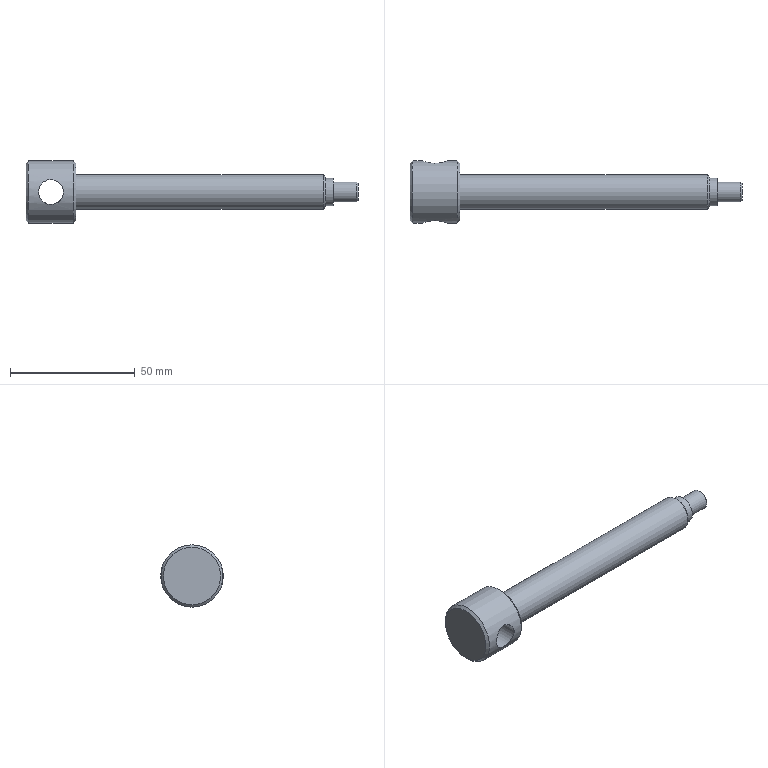Component | NX | SCREW_ROD | 1 solid | 14 faces | box 133 x 25 x 25 mm | volume 23976 mm3 | cylinder 5 | plane 5 | cone 4 | commonest cylinder face diameters 25 x1 8 x1 11 x1 14 x1 10 x1
STEP:
#1=CARTESIAN_POINT('',(0.,0.,0.));
#2=DIRECTION('',(0.,0.,1.));
#3=DIRECTION('',(1.,0.,0.));
#4=AXIS2_PLACEMENT_3D('',#1,#2,#3);
#5=CARTESIAN_POINT('',(-201.627,0.,27.5));
#6=VERTEX_POINT('',#5);
#7=CARTESIAN_POINT('',(-201.627,0.,15.));
#8=DIRECTION('',(1.,0.,0.));
#9=DIRECTION('',(0.,0.,1.));
#10=AXIS2_PLACEMENT_3D('',#7,#8,#9);
#11=CIRCLE('',#10,12.5);
#12=CARTESIAN_POINT('',(-182.627,0.,15.));
#13=DIRECTION('',(-1.,0.,0.));
#14=DIRECTION('',(0.,0.,1.));
#15=AXIS2_PLACEMENT_3D('',#12,#13,#14);
#16=CYLINDRICAL_SURFACE('',#15,12.5);
#17=CARTESIAN_POINT('',(6.283,19.));
#18=DIRECTION('',(-1.,0.));
#19=VECTOR('',#18,1.);
#20=LINE('',#17,#19);
#21=(GEOMETRIC_REPRESENTATION_CONTEXT(2)PARAMETRIC_REPRESENTATION_CONTEXT()REPRESENTATION_CONTEXT('',''));
#22=DEFINITIONAL_REPRESENTATION('',(#20),#21);
#23=PCURVE('',#16,#22);
#24=CARTESIAN_POINT('',(-201.627,0.,15.));
#25=DIRECTION('',(1.,0.,0.));
#26=DIRECTION('',(0.,0.,-1.));
#27=AXIS2_PLACEMENT_3D('',#24,#25,#26);
#28=CONICAL_SURFACE('',#27,12.5,0.7854);
#29=CARTESIAN_POINT('',(3.142,0.));
#30=DIRECTION('',(1.,0.));
#31=VECTOR('',#30,1.);
#32=LINE('',#29,#31);
#33=(GEOMETRIC_REPRESENTATION_CONTEXT(2)PARAMETRIC_REPRESENTATION_CONTEXT()REPRESENTATION_CONTEXT('',''));
#34=DEFINITIONAL_REPRESENTATION('',(#32),#33);
#35=PCURVE('',#28,#34);
#36=SURFACE_CURVE('',#11,(#23,#35),.PCURVE_S1.);
#37=EDGE_CURVE('',#6,#6,#36,.T.);
#38=ORIENTED_EDGE('',*,*,#37,.T.);
#39=CARTESIAN_POINT('',(-183.627,-0.,27.5));
#40=VERTEX_POINT('',#39);
#41=CARTESIAN_POINT('',(-183.627,-0.,27.5));
#42=CARTESIAN_POINT('',(-201.627,-0.,27.5));
#43=B_SPLINE_CURVE_WITH_KNOTS('',1,(#41,#42),.UNSPECIFIED.,.F.,.F.,(2,2),(1.,19.),.PIECEWISE_BEZIER_KNOTS.);
#44=CARTESIAN_POINT('',(0.,0.));
#45=DIRECTION('',(0.,1.));
#46=VECTOR('',#45,1.);
#47=LINE('',#44,#46);
#48=(GEOMETRIC_REPRESENTATION_CONTEXT(2)PARAMETRIC_REPRESENTATION_CONTEXT()REPRESENTATION_CONTEXT('',''));
#49=DEFINITIONAL_REPRESENTATION('',(#47),#48);
#50=PCURVE('',#16,#49);
#51=CARTESIAN_POINT('',(6.283,0.));
#52=DIRECTION('',(0.,1.));
#53=VECTOR('',#52,1.);
#54=LINE('',#51,#53);
#55=(GEOMETRIC_REPRESENTATION_CONTEXT(2)PARAMETRIC_REPRESENTATION_CONTEXT()REPRESENTATION_CONTEXT('',''));
#56=DEFINITIONAL_REPRESENTATION('',(#54),#55);
#57=PCURVE('',#16,#56);
#58=SEAM_CURVE('',#43,(#50,#57),.PCURVE_S1.);
#59=EDGE_CURVE('',#40,#6,#58,.T.);
#60=ORIENTED_EDGE('',*,*,#59,.F.);
#61=CARTESIAN_POINT('',(-183.627,0.,2.5));
#62=VERTEX_POINT('',#61);
#63=CARTESIAN_POINT('',(-183.627,0.,15.));
#64=DIRECTION('',(-1.,0.,0.));
#65=DIRECTION('',(0.,0.,-1.));
#66=AXIS2_PLACEMENT_3D('',#63,#64,#65);
#67=CIRCLE('',#66,12.5);
#68=CARTESIAN_POINT('',(-3.142,1.));
#69=DIRECTION('',(1.,0.));
#70=VECTOR('',#69,1.);
#71=LINE('',#68,#70);
#72=(GEOMETRIC_REPRESENTATION_CONTEXT(2)PARAMETRIC_REPRESENTATION_CONTEXT()REPRESENTATION_CONTEXT('',''));
#73=DEFINITIONAL_REPRESENTATION('',(#71),#72);
#74=PCURVE('',#16,#73);
#75=CARTESIAN_POINT('',(-183.627,0.,15.));
#76=DIRECTION('',(-1.,0.,0.));
#77=DIRECTION('',(0.,0.,1.));
#78=AXIS2_PLACEMENT_3D('',#75,#76,#77);
#79=CONICAL_SURFACE('',#78,12.5,0.7854);
#80=CARTESIAN_POINT('',(3.142,0.));
#81=DIRECTION('',(1.,0.));
#82=VECTOR('',#81,1.);
#83=LINE('',#80,#82);
#84=(GEOMETRIC_REPRESENTATION_CONTEXT(2)PARAMETRIC_REPRESENTATION_CONTEXT()REPRESENTATION_CONTEXT('',''));
#85=DEFINITIONAL_REPRESENTATION('',(#83),#84);
#86=PCURVE('',#79,#85);
#87=SURFACE_CURVE('',#67,(#74,#86),.PCURVE_S1.);
#88=EDGE_CURVE('',#40,#62,#87,.T.);
#89=ORIENTED_EDGE('',*,*,#88,.T.);
#90=CARTESIAN_POINT('',(-183.627,0.,15.));
#91=DIRECTION('',(-1.,0.,0.));
#92=DIRECTION('',(0.,0.,-1.));
#93=AXIS2_PLACEMENT_3D('',#90,#91,#92);
#94=CIRCLE('',#93,12.5);
#95=CARTESIAN_POINT('',(3.142,1.));
#96=DIRECTION('',(1.,0.));
#97=VECTOR('',#96,1.);
#98=LINE('',#95,#97);
#99=(GEOMETRIC_REPRESENTATION_CONTEXT(2)PARAMETRIC_REPRESENTATION_CONTEXT()REPRESENTATION_CONTEXT('',''));
#100=DEFINITIONAL_REPRESENTATION('',(#98),#99);
#101=PCURVE('',#16,#100);
#102=CARTESIAN_POINT('',(3.142,0.));
#103=DIRECTION('',(1.,0.));
#104=VECTOR('',#103,1.);
#105=LINE('',#102,#104);
#106=(GEOMETRIC_REPRESENTATION_CONTEXT(2)PARAMETRIC_REPRESENTATION_CONTEXT()REPRESENTATION_CONTEXT('',''));
#107=DEFINITIONAL_REPRESENTATION('',(#105),#106);
#108=PCURVE('',#79,#107);
#109=SURFACE_CURVE('',#94,(#101,#108),.PCURVE_S1.);
#110=EDGE_CURVE('',#62,#40,#109,.T.);
#111=ORIENTED_EDGE('',*,*,#110,.T.);
#112=ORIENTED_EDGE('',*,*,#59,.T.);
#113=EDGE_LOOP('',(#38,#60,#89,#111,#112));
#114=FACE_BOUND('',#113,.T.);
#115=CARTESIAN_POINT('',(-197.627,12.5,15.));
#116=VERTEX_POINT('',#115);
#117=CARTESIAN_POINT('',(-197.627,12.5,16.336));
#118=CARTESIAN_POINT('',(-197.627,12.5,13.664));
#119=CARTESIAN_POINT('',(-197.074,12.258,12.375));
#120=CARTESIAN_POINT('',(-195.249,11.72,10.551));
#121=CARTESIAN_POINT('',(-193.953,11.457,10.001));
#122=CARTESIAN_POINT('',(-191.313,11.456,9.999));
#123=CARTESIAN_POINT('',(-190.009,11.719,10.548));
#124=CARTESIAN_POINT('',(-188.178,12.259,12.378));
#125=CARTESIAN_POINT('',(-187.629,12.499,13.679));
#126=CARTESIAN_POINT('',(-187.626,12.501,16.311));
#127=CARTESIAN_POINT('',(-188.169,12.262,17.613));
#128=CARTESIAN_POINT('',(-190.015,11.717,19.458));
#129=CARTESIAN_POINT('',(-191.306,11.457,19.999));
#130=CARTESIAN_POINT('',(-193.943,11.456,20.001));
#131=CARTESIAN_POINT('',(-195.242,11.718,19.455));
#132=CARTESIAN_POINT('',(-197.079,12.259,17.621));
#133=CARTESIAN_POINT('',(-197.627,12.5,16.336));
#134=CARTESIAN_POINT('',(-197.627,12.5,13.664));
#135=B_SPLINE_CURVE_WITH_KNOTS('',3,(#117,#118,#119,#120,#121,#122,#123,#124,#125,#126,#127,#128,#129,#130,#131,#132,#133,#134),.UNSPECIFIED.,.T.,.F.,(2,2,2,2,2,2,2,2,2,2,2),(-0.125,0.,0.125,0.25,0.375,0.5,0.625,0.75,0.875,1.,1.125),.UNSPECIFIED.);
#136=CARTESIAN_POINT('',(1.571,15.));
#137=CARTESIAN_POINT('',(1.59,15.));
#138=CARTESIAN_POINT('',(1.629,14.963));
#139=CARTESIAN_POINT('',(1.685,14.806));
#140=CARTESIAN_POINT('',(1.739,14.552));
#141=CARTESIAN_POINT('',(1.79,14.21));
#142=CARTESIAN_POINT('',(1.837,13.786));
#143=CARTESIAN_POINT('',(1.879,13.288));
#144=CARTESIAN_POINT('',(1.914,12.719));
#145=CARTESIAN_POINT('',(1.943,12.093));
#146=CARTESIAN_POINT('',(1.965,11.424));
#147=CARTESIAN_POINT('',(1.979,10.724));
#148=CARTESIAN_POINT('',(1.984,10.006));
#149=CARTESIAN_POINT('',(1.979,9.287));
#150=CARTESIAN_POINT('',(1.965,8.585));
#151=CARTESIAN_POINT('',(1.944,7.913));
#152=CARTESIAN_POINT('',(1.915,7.285));
#153=CARTESIAN_POINT('',(1.879,6.713));
#154=CARTESIAN_POINT('',(1.837,6.213));
#155=CARTESIAN_POINT('',(1.79,5.789));
#156=CARTESIAN_POINT('',(1.739,5.447));
#157=CARTESIAN_POINT('',(1.685,5.194));
#158=CARTESIAN_POINT('',(1.629,5.037));
#159=CARTESIAN_POINT('',(1.571,4.982));
#160=CARTESIAN_POINT('',(1.514,5.035));
#161=CARTESIAN_POINT('',(1.458,5.19));
#162=CARTESIAN_POINT('',(1.403,5.442));
#163=CARTESIAN_POINT('',(1.352,5.783));
#164=CARTESIAN_POINT('',(1.305,6.209));
#165=CARTESIAN_POINT('',(1.263,6.714));
#166=CARTESIAN_POINT('',(1.227,7.286));
#167=CARTESIAN_POINT('',(1.198,7.912));
#168=CARTESIAN_POINT('',(1.176,8.581));
#169=CARTESIAN_POINT('',(1.162,9.279));
#170=CARTESIAN_POINT('',(1.158,9.997));
#171=CARTESIAN_POINT('',(1.162,10.715));
#172=CARTESIAN_POINT('',(1.176,11.415));
#173=CARTESIAN_POINT('',(1.198,12.086));
#174=CARTESIAN_POINT('',(1.227,12.713));
#175=CARTESIAN_POINT('',(1.263,13.285));
#176=CARTESIAN_POINT('',(1.305,13.787));
#177=CARTESIAN_POINT('',(1.351,14.212));
#178=CARTESIAN_POINT('',(1.402,14.554));
#179=CARTESIAN_POINT('',(1.456,14.807));
#180=CARTESIAN_POINT('',(1.513,14.964));
#181=CARTESIAN_POINT('',(1.551,15.));
#182=CARTESIAN_POINT('',(1.571,15.));
#183=B_SPLINE_CURVE_WITH_KNOTS('',3,(#136,#137,#138,#139,#140,#141,#142,#143,#144,#145,#146,#147,#148,#149,#150,#151,#152,#153,#154,#155,#156,#157,#158,#159,#160,#161,#162,#163,#164,#165,#166,#167,#168,#169,#170,#171,#172,#173,#174,#175,#176,#177,#178,#179,#180,#181,#182),.UNSPECIFIED.,.T.,.F.,(4,1,1,1,1,1,1,1,1,1,1,1,1,1,1,1,1,1,1,1,1,1,1,1,1,1,1,1,1,1,1,1,1,1,1,1,1,1,1,1,1,1,1,1,4),(0.,0.02273,0.04545,0.06818,0.09091,0.1136,0.1364,0.1591,0.1818,0.2045,0.2273,0.25,0.2727,0.2955,0.3182,0.3409,0.3636,0.3864,0.4091,0.4318,0.4545,0.4773,0.5,0.5227,0.5455,0.5682,0.5909,0.6136,0.6364,0.6591,0.6818,0.7045,0.7273,0.75,0.7727,0.7955,0.8182,0.8409,0.8636,0.8864,0.9091,0.9318,0.9545,0.9773,1.),.QUASI_UNIFORM_KNOTS.);
#184=(GEOMETRIC_REPRESENTATION_CONTEXT(2)PARAMETRIC_REPRESENTATION_CONTEXT()REPRESENTATION_CONTEXT('',''));
#185=DEFINITIONAL_REPRESENTATION('',(#183),#184);
#186=PCURVE('',#16,#185);
#187=CARTESIAN_POINT('',(-192.627,-30.,15.));
#188=DIRECTION('',(0.,1.,0.));
#189=DIRECTION('',(-1.,0.,0.));
#190=AXIS2_PLACEMENT_3D('',#187,#188,#189);
#191=CYLINDRICAL_SURFACE('',#190,5.);
#192=CARTESIAN_POINT('',(6.283,42.5));
#193=CARTESIAN_POINT('',(6.235,42.5));
#194=CARTESIAN_POINT('',(6.138,42.484));
#195=CARTESIAN_POINT('',(5.994,42.42));
#196=CARTESIAN_POINT('',(5.851,42.323));
#197=CARTESIAN_POINT('',(5.709,42.202));
#198=CARTESIAN_POINT('',(5.568,42.063));
#199=CARTESIAN_POINT('',(5.427,41.915));
#200=CARTESIAN_POINT('',(5.286,41.773));
#201=CARTESIAN_POINT('',(5.143,41.646));
#202=CARTESIAN_POINT('',(5.,41.543));
#203=CARTESIAN_POINT('',(4.857,41.474));
#204=CARTESIAN_POINT('',(4.714,41.448));
#205=CARTESIAN_POINT('',(4.57,41.474));
#206=CARTESIAN_POINT('',(4.426,41.543));
#207=CARTESIAN_POINT('',(4.283,41.645));
#208=CARTESIAN_POINT('',(4.14,41.773));
#209=CARTESIAN_POINT('',(3.998,41.915));
#210=CARTESIAN_POINT('',(3.857,42.064));
#211=CARTESIAN_POINT('',(3.715,42.202));
#212=CARTESIAN_POINT('',(3.572,42.323));
#213=CARTESIAN_POINT('',(3.429,42.42));
#214=CARTESIAN_POINT('',(3.286,42.484));
#215=CARTESIAN_POINT('',(3.143,42.508));
#216=CARTESIAN_POINT('',(2.999,42.484));
#217=CARTESIAN_POINT('',(2.856,42.421));
#218=CARTESIAN_POINT('',(2.713,42.325));
#219=CARTESIAN_POINT('',(2.57,42.204));
#220=CARTESIAN_POINT('',(2.427,42.065));
#221=CARTESIAN_POINT('',(2.285,41.915));
#222=CARTESIAN_POINT('',(2.143,41.772));
#223=CARTESIAN_POINT('',(2.,41.645));
#224=CARTESIAN_POINT('',(1.858,41.543));
#225=CARTESIAN_POINT('',(1.715,41.474));
#226=CARTESIAN_POINT('',(1.571,41.448));
#227=CARTESIAN_POINT('',(1.428,41.474));
#228=CARTESIAN_POINT('',(1.285,41.542));
#229=CARTESIAN_POINT('',(1.142,41.645));
#230=CARTESIAN_POINT('',(0.9989,41.772));
#231=CARTESIAN_POINT('',(0.8569,41.914));
#232=CARTESIAN_POINT('',(0.7153,42.064));
#233=CARTESIAN_POINT('',(0.5736,42.202));
#234=CARTESIAN_POINT('',(0.4314,42.324));
#235=CARTESIAN_POINT('',(0.2887,42.42));
#236=CARTESIAN_POINT('',(0.1451,42.484));
#237=CARTESIAN_POINT('',(0.04856,42.5));
#238=CARTESIAN_POINT('',(0.,42.5));
#239=B_SPLINE_CURVE_WITH_KNOTS('',3,(#192,#193,#194,#195,#196,#197,#198,#199,#200,#201,#202,#203,#204,#205,#206,#207,#208,#209,#210,#211,#212,#213,#214,#215,#216,#217,#218,#219,#220,#221,#222,#223,#224,#225,#226,#227,#228,#229,#230,#231,#232,#233,#234,#235,#236,#237,#238),.UNSPECIFIED.,.F.,.F.,(4,1,1,1,1,1,1,1,1,1,1,1,1,1,1,1,1,1,1,1,1,1,1,1,1,1,1,1,1,1,1,1,1,1,1,1,1,1,1,1,1,1,1,1,4),(0.,0.02273,0.04545,0.06818,0.09091,0.1136,0.1364,0.1591,0.1818,0.2045,0.2273,0.25,0.2727,0.2955,0.3182,0.3409,0.3636,0.3864,0.4091,0.4318,0.4545,0.4773,0.5,0.5227,0.5455,0.5682,0.5909,0.6136,0.6364,0.6591,0.6818,0.7045,0.7273,0.75,0.7727,0.7955,0.8182,0.8409,0.8636,0.8864,0.9091,0.9318,0.9545,0.9773,1.),.QUASI_UNIFORM_KNOTS.);
#240=(GEOMETRIC_REPRESENTATION_CONTEXT(2)PARAMETRIC_REPRESENTATION_CONTEXT()REPRESENTATION_CONTEXT('',''));
#241=DEFINITIONAL_REPRESENTATION('',(#239),#240);
#242=PCURVE('',#191,#241);
#243=SURFACE_CURVE('',#135,(#186,#242),.PCURVE_S1.);
#244=EDGE_CURVE('',#116,#116,#243,.T.);
#245=ORIENTED_EDGE('',*,*,#244,.T.);
#246=EDGE_LOOP('',(#245));
#247=FACE_BOUND('',#246,.T.);
#248=CARTESIAN_POINT('',(-197.627,-12.5,15.));
#249=VERTEX_POINT('',#248);
#250=CARTESIAN_POINT('',(-197.627,-12.5,13.664));
#251=CARTESIAN_POINT('',(-197.627,-12.5,16.336));
#252=CARTESIAN_POINT('',(-197.074,-12.258,17.625));
#253=CARTESIAN_POINT('',(-195.249,-11.72,19.449));
#254=CARTESIAN_POINT('',(-193.953,-11.457,19.999));
#255=CARTESIAN_POINT('',(-191.313,-11.456,20.001));
#256=CARTESIAN_POINT('',(-190.009,-11.719,19.452));
#257=CARTESIAN_POINT('',(-188.178,-12.259,17.622));
#258=CARTESIAN_POINT('',(-187.629,-12.499,16.321));
#259=CARTESIAN_POINT('',(-187.626,-12.501,13.689));
#260=CARTESIAN_POINT('',(-188.169,-12.262,12.387));
#261=CARTESIAN_POINT('',(-190.015,-11.717,10.542));
#262=CARTESIAN_POINT('',(-191.306,-11.457,10.001));
#263=CARTESIAN_POINT('',(-193.943,-11.456,9.999));
#264=CARTESIAN_POINT('',(-195.242,-11.718,10.545));
#265=CARTESIAN_POINT('',(-197.079,-12.259,12.379));
#266=CARTESIAN_POINT('',(-197.627,-12.5,13.664));
#267=CARTESIAN_POINT('',(-197.627,-12.5,16.336));
#268=B_SPLINE_CURVE_WITH_KNOTS('',3,(#250,#251,#252,#253,#254,#255,#256,#257,#258,#259,#260,#261,#262,#263,#264,#265,#266,#267),.UNSPECIFIED.,.T.,.F.,(2,2,2,2,2,2,2,2,2,2,2),(-0.125,0.,0.125,0.25,0.375,0.5,0.625,0.75,0.875,1.,1.125),.UNSPECIFIED.);
#269=CARTESIAN_POINT('',(4.712,15.));
#270=CARTESIAN_POINT('',(4.732,15.));
#271=CARTESIAN_POINT('',(4.77,14.963));
#272=CARTESIAN_POINT('',(4.827,14.806));
#273=CARTESIAN_POINT('',(4.881,14.552));
#274=CARTESIAN_POINT('',(4.932,14.21));
#275=CARTESIAN_POINT('',(4.979,13.786));
#276=CARTESIAN_POINT('',(5.02,13.288));
#277=CARTESIAN_POINT('',(5.056,12.719));
#278=CARTESIAN_POINT('',(5.085,12.093));
#279=CARTESIAN_POINT('',(5.107,11.424));
#280=CARTESIAN_POINT('',(5.121,10.724));
#281=CARTESIAN_POINT('',(5.126,10.006));
#282=CARTESIAN_POINT('',(5.121,9.287));
#283=CARTESIAN_POINT('',(5.107,8.585));
#284=CARTESIAN_POINT('',(5.085,7.913));
#285=CARTESIAN_POINT('',(5.056,7.285));
#286=CARTESIAN_POINT('',(5.02,6.713));
#287=CARTESIAN_POINT('',(4.979,6.213));
#288=CARTESIAN_POINT('',(4.932,5.789));
#289=CARTESIAN_POINT('',(4.881,5.447));
#290=CARTESIAN_POINT('',(4.826,5.194));
#291=CARTESIAN_POINT('',(4.77,5.037));
#292=CARTESIAN_POINT('',(4.713,4.982));
#293=CARTESIAN_POINT('',(4.655,5.035));
#294=CARTESIAN_POINT('',(4.599,5.19));
#295=CARTESIAN_POINT('',(4.545,5.442));
#296=CARTESIAN_POINT('',(4.494,5.783));
#297=CARTESIAN_POINT('',(4.446,6.209));
#298=CARTESIAN_POINT('',(4.404,6.714));
#299=CARTESIAN_POINT('',(4.368,7.286));
#300=CARTESIAN_POINT('',(4.339,7.912));
#301=CARTESIAN_POINT('',(4.318,8.581));
#302=CARTESIAN_POINT('',(4.304,9.279));
#303=CARTESIAN_POINT('',(4.299,9.997));
#304=CARTESIAN_POINT('',(4.304,10.715));
#305=CARTESIAN_POINT('',(4.318,11.415));
#306=CARTESIAN_POINT('',(4.339,12.086));
#307=CARTESIAN_POINT('',(4.368,12.713));
#308=CARTESIAN_POINT('',(4.404,13.285));
#309=CARTESIAN_POINT('',(4.446,13.787));
#310=CARTESIAN_POINT('',(4.493,14.212));
#311=CARTESIAN_POINT('',(4.544,14.554));
#312=CARTESIAN_POINT('',(4.598,14.807));
#313=CARTESIAN_POINT('',(4.654,14.964));
#314=CARTESIAN_POINT('',(4.693,15.));
#315=CARTESIAN_POINT('',(4.712,15.));
#316=B_SPLINE_CURVE_WITH_KNOTS('',3,(#269,#270,#271,#272,#273,#274,#275,#276,#277,#278,#279,#280,#281,#282,#283,#284,#285,#286,#287,#288,#289,#290,#291,#292,#293,#294,#295,#296,#297,#298,#299,#300,#301,#302,#303,#304,#305,#306,#307,#308,#309,#310,#311,#312,#313,#314,#315),.UNSPECIFIED.,.T.,.F.,(4,1,1,1,1,1,1,1,1,1,1,1,1,1,1,1,1,1,1,1,1,1,1,1,1,1,1,1,1,1,1,1,1,1,1,1,1,1,1,1,1,1,1,1,4),(0.,0.02273,0.04545,0.06818,0.09091,0.1136,0.1364,0.1591,0.1818,0.2045,0.2273,0.25,0.2727,0.2955,0.3182,0.3409,0.3636,0.3864,0.4091,0.4318,0.4545,0.4773,0.5,0.5227,0.5455,0.5682,0.5909,0.6136,0.6364,0.6591,0.6818,0.7045,0.7273,0.75,0.7727,0.7955,0.8182,0.8409,0.8636,0.8864,0.9091,0.9318,0.9545,0.9773,1.),.QUASI_UNIFORM_KNOTS.);
#317=(GEOMETRIC_REPRESENTATION_CONTEXT(2)PARAMETRIC_REPRESENTATION_CONTEXT()REPRESENTATION_CONTEXT('',''));
#318=DEFINITIONAL_REPRESENTATION('',(#316),#317);
#319=PCURVE('',#16,#318);
#320=CARTESIAN_POINT('',(0.,17.5));
#321=CARTESIAN_POINT('',(0.04855,17.5));
#322=CARTESIAN_POINT('',(0.1452,17.516));
#323=CARTESIAN_POINT('',(0.2889,17.58));
#324=CARTESIAN_POINT('',(0.4319,17.677));
#325=CARTESIAN_POINT('',(0.5741,17.798));
#326=CARTESIAN_POINT('',(0.7155,17.937));
#327=CARTESIAN_POINT('',(0.8561,18.085));
#328=CARTESIAN_POINT('',(0.9976,18.227));
#329=CARTESIAN_POINT('',(1.14,18.354));
#330=CARTESIAN_POINT('',(1.283,18.457));
#331=CARTESIAN_POINT('',(1.426,18.526));
#332=CARTESIAN_POINT('',(1.57,18.552));
#333=CARTESIAN_POINT('',(1.714,18.526));
#334=CARTESIAN_POINT('',(1.857,18.457));
#335=CARTESIAN_POINT('',(2.,18.355));
#336=CARTESIAN_POINT('',(2.143,18.227));
#337=CARTESIAN_POINT('',(2.285,18.085));
#338=CARTESIAN_POINT('',(2.426,17.936));
#339=CARTESIAN_POINT('',(2.568,17.798));
#340=CARTESIAN_POINT('',(2.711,17.677));
#341=CARTESIAN_POINT('',(2.854,17.58));
#342=CARTESIAN_POINT('',(2.997,17.516));
#343=CARTESIAN_POINT('',(3.141,17.492));
#344=CARTESIAN_POINT('',(3.284,17.516));
#345=CARTESIAN_POINT('',(3.427,17.579));
#346=CARTESIAN_POINT('',(3.57,17.675));
#347=CARTESIAN_POINT('',(3.713,17.796));
#348=CARTESIAN_POINT('',(3.856,17.935));
#349=CARTESIAN_POINT('',(3.998,18.085));
#350=CARTESIAN_POINT('',(4.14,18.228));
#351=CARTESIAN_POINT('',(4.283,18.355));
#352=CARTESIAN_POINT('',(4.425,18.457));
#353=CARTESIAN_POINT('',(4.568,18.526));
#354=CARTESIAN_POINT('',(4.712,18.552));
#355=CARTESIAN_POINT('',(4.855,18.526));
#356=CARTESIAN_POINT('',(4.999,18.458));
#357=CARTESIAN_POINT('',(5.142,18.355));
#358=CARTESIAN_POINT('',(5.284,18.228));
#359=CARTESIAN_POINT('',(5.426,18.086));
#360=CARTESIAN_POINT('',(5.568,17.936));
#361=CARTESIAN_POINT('',(5.71,17.798));
#362=CARTESIAN_POINT('',(5.852,17.676));
#363=CARTESIAN_POINT('',(5.995,17.58));
#364=CARTESIAN_POINT('',(6.138,17.516));
#365=CARTESIAN_POINT('',(6.235,17.5));
#366=CARTESIAN_POINT('',(6.283,17.5));
#367=B_SPLINE_CURVE_WITH_KNOTS('',3,(#320,#321,#322,#323,#324,#325,#326,#327,#328,#329,#330,#331,#332,#333,#334,#335,#336,#337,#338,#339,#340,#341,#342,#343,#344,#345,#346,#347,#348,#349,#350,#351,#352,#353,#354,#355,#356,#357,#358,#359,#360,#361,#362,#363,#364,#365,#366),.UNSPECIFIED.,.F.,.F.,(4,1,1,1,1,1,1,1,1,1,1,1,1,1,1,1,1,1,1,1,1,1,1,1,1,1,1,1,1,1,1,1,1,1,1,1,1,1,1,1,1,1,1,1,4),(0.,0.02273,0.04545,0.06818,0.09091,0.1136,0.1364,0.1591,0.1818,0.2045,0.2273,0.25,0.2727,0.2955,0.3182,0.3409,0.3636,0.3864,0.4091,0.4318,0.4545,0.4773,0.5,0.5227,0.5455,0.5682,0.5909,0.6136,0.6364,0.6591,0.6818,0.7045,0.7273,0.75,0.7727,0.7955,0.8182,0.8409,0.8636,0.8864,0.9091,0.9318,0.9545,0.9773,1.),.QUASI_UNIFORM_KNOTS.);
#368=(GEOMETRIC_REPRESENTATION_CONTEXT(2)PARAMETRIC_REPRESENTATION_CONTEXT()REPRESENTATION_CONTEXT('',''));
#369=DEFINITIONAL_REPRESENTATION('',(#367),#368);
#370=PCURVE('',#191,#369);
#371=SURFACE_CURVE('',#268,(#319,#370),.PCURVE_S1.);
#372=EDGE_CURVE('',#249,#249,#371,.T.);
#373=ORIENTED_EDGE('',*,*,#372,.T.);
#374=EDGE_LOOP('',(#373));
#375=FACE_BOUND('',#374,.T.);
#376=ADVANCED_FACE('',(#114,#247,#375),#16,.T.);
#377=CARTESIAN_POINT('',(-69.627,0.,11.5));
#378=VERTEX_POINT('',#377);
#379=CARTESIAN_POINT('',(-69.627,0.,15.));
#380=DIRECTION('',(1.,0.,0.));
#381=DIRECTION('',(0.,0.,-1.));
#382=AXIS2_PLACEMENT_3D('',#379,#380,#381);
#383=CIRCLE('',#382,3.5);
#384=CARTESIAN_POINT('',(-69.627,0.,15.));
#385=DIRECTION('',(1.,0.,0.));
#386=DIRECTION('',(0.,0.,-1.));
#387=AXIS2_PLACEMENT_3D('',#384,#385,#386);
#388=PLANE('',#387);
#389=CARTESIAN_POINT('',(0.,0.));
#390=DIRECTION('',(1.,0.));
#391=AXIS2_PLACEMENT_2D('',#389,#390);
#392=CIRCLE('',#391,3.5);
#393=(GEOMETRIC_REPRESENTATION_CONTEXT(2)PARAMETRIC_REPRESENTATION_CONTEXT()REPRESENTATION_CONTEXT('',''));
#394=DEFINITIONAL_REPRESENTATION('',(#392),#393);
#395=PCURVE('',#388,#394);
#396=CARTESIAN_POINT('',(-70.127,0.,15.));
#397=DIRECTION('',(-1.,0.,0.));
#398=DIRECTION('',(0.,0.,1.));
#399=AXIS2_PLACEMENT_3D('',#396,#397,#398);
#400=CONICAL_SURFACE('',#399,4.,0.7854);
#401=CARTESIAN_POINT('',(9.425,-0.5));
#402=DIRECTION('',(-1.,0.));
#403=VECTOR('',#402,1.);
#404=LINE('',#401,#403);
#405=(GEOMETRIC_REPRESENTATION_CONTEXT(2)PARAMETRIC_REPRESENTATION_CONTEXT()REPRESENTATION_CONTEXT('',''));
#406=DEFINITIONAL_REPRESENTATION('',(#404),#405);
#407=PCURVE('',#400,#406);
#408=SURFACE_CURVE('',#383,(#395,#407),.PCURVE_S1.);
#409=EDGE_CURVE('',#378,#378,#408,.T.);
#410=ORIENTED_EDGE('',*,*,#409,.T.);
#411=EDGE_LOOP('',(#410));
#412=FACE_BOUND('',#411,.T.);
#413=ADVANCED_FACE('',(#412),#388,.T.);
#414=CARTESIAN_POINT('',(-70.127,0.,11.));
#415=VERTEX_POINT('',#414);
#416=CARTESIAN_POINT('',(-70.127,0.,15.));
#417=DIRECTION('',(-1.,0.,0.));
#418=DIRECTION('',(0.,0.,-1.));
#419=AXIS2_PLACEMENT_3D('',#416,#417,#418);
#420=CIRCLE('',#419,4.);
#421=CARTESIAN_POINT('',(-69.627,0.,15.));
#422=DIRECTION('',(-1.,0.,0.));
#423=DIRECTION('',(0.,0.,1.));
#424=AXIS2_PLACEMENT_3D('',#421,#422,#423);
#425=CYLINDRICAL_SURFACE('',#424,4.);
#426=CARTESIAN_POINT('',(3.142,0.5));
#427=DIRECTION('',(1.,0.));
#428=VECTOR('',#427,1.);
#429=LINE('',#426,#428);
#430=(GEOMETRIC_REPRESENTATION_CONTEXT(2)PARAMETRIC_REPRESENTATION_CONTEXT()REPRESENTATION_CONTEXT('',''));
#431=DEFINITIONAL_REPRESENTATION('',(#429),#430);
#432=PCURVE('',#425,#431);
#433=CARTESIAN_POINT('',(3.142,0.));
#434=DIRECTION('',(1.,0.));
#435=VECTOR('',#434,1.);
#436=LINE('',#433,#435);
#437=(GEOMETRIC_REPRESENTATION_CONTEXT(2)PARAMETRIC_REPRESENTATION_CONTEXT()REPRESENTATION_CONTEXT('',''));
#438=DEFINITIONAL_REPRESENTATION('',(#436),#437);
#439=PCURVE('',#400,#438);
#440=SURFACE_CURVE('',#420,(#432,#439),.PCURVE_S1.);
#441=EDGE_CURVE('',#415,#415,#440,.T.);
#442=ORIENTED_EDGE('',*,*,#441,.T.);
#443=CARTESIAN_POINT('',(-79.627,0.,11.));
#444=VERTEX_POINT('',#443);
#445=CARTESIAN_POINT('',(-70.127,0.,11.));
#446=CARTESIAN_POINT('',(-79.627,0.,11.));
#447=B_SPLINE_CURVE_WITH_KNOTS('',1,(#445,#446),.UNSPECIFIED.,.F.,.F.,(2,2),(0.5,10.),.PIECEWISE_BEZIER_KNOTS.);
#448=CARTESIAN_POINT('',(9.425,0.));
#449=DIRECTION('',(0.,1.));
#450=VECTOR('',#449,1.);
#451=LINE('',#448,#450);
#452=(GEOMETRIC_REPRESENTATION_CONTEXT(2)PARAMETRIC_REPRESENTATION_CONTEXT()REPRESENTATION_CONTEXT('',''));
#453=DEFINITIONAL_REPRESENTATION('',(#451),#452);
#454=PCURVE('',#425,#453);
#455=CARTESIAN_POINT('',(3.142,0.));
#456=DIRECTION('',(0.,1.));
#457=VECTOR('',#456,1.);
#458=LINE('',#455,#457);
#459=(GEOMETRIC_REPRESENTATION_CONTEXT(2)PARAMETRIC_REPRESENTATION_CONTEXT()REPRESENTATION_CONTEXT('',''));
#460=DEFINITIONAL_REPRESENTATION('',(#458),#459);
#461=PCURVE('',#425,#460);
#462=SEAM_CURVE('',#447,(#454,#461),.PCURVE_S1.);
#463=EDGE_CURVE('',#415,#444,#462,.T.);
#464=ORIENTED_EDGE('',*,*,#463,.T.);
#465=CARTESIAN_POINT('',(-79.627,0.,15.));
#466=DIRECTION('',(-1.,0.,0.));
#467=DIRECTION('',(0.,0.,-1.));
#468=AXIS2_PLACEMENT_3D('',#465,#466,#467);
#469=CIRCLE('',#468,4.);
#470=CARTESIAN_POINT('',(3.142,10.));
#471=DIRECTION('',(1.,0.));
#472=VECTOR('',#471,1.);
#473=LINE('',#470,#472);
#474=(GEOMETRIC_REPRESENTATION_CONTEXT(2)PARAMETRIC_REPRESENTATION_CONTEXT()REPRESENTATION_CONTEXT('',''));
#475=DEFINITIONAL_REPRESENTATION('',(#473),#474);
#476=PCURVE('',#425,#475);
#477=CARTESIAN_POINT('',(-79.627,0.,15.));
#478=DIRECTION('',(1.,0.,0.));
#479=DIRECTION('',(0.,0.,-1.));
#480=AXIS2_PLACEMENT_3D('',#477,#478,#479);
#481=PLANE('',#480);
#482=CARTESIAN_POINT('',(4.,0.));
#483=CARTESIAN_POINT('',(4.,-6.928));
#484=CARTESIAN_POINT('',(-2.,-3.464));
#485=CARTESIAN_POINT('',(-8.,-0.));
#486=CARTESIAN_POINT('',(-2.,3.464));
#487=CARTESIAN_POINT('',(4.,6.928));
#488=CARTESIAN_POINT('',(4.,0.));
#489=(BOUNDED_CURVE()B_SPLINE_CURVE(2,(#482,#483,#484,#485,#486,#487,#488),.UNSPECIFIED.,.T.,.F.)B_SPLINE_CURVE_WITH_KNOTS((1,2,2,2,2,1),(-2.094,0.,2.094,4.189,6.283,8.378),.UNSPECIFIED.)CURVE()GEOMETRIC_REPRESENTATION_ITEM()RATIONAL_B_SPLINE_CURVE((1.,0.5,1.,0.5,1.,0.5,1.))REPRESENTATION_ITEM(''));
#490=(GEOMETRIC_REPRESENTATION_CONTEXT(2)PARAMETRIC_REPRESENTATION_CONTEXT()REPRESENTATION_CONTEXT('',''));
#491=DEFINITIONAL_REPRESENTATION('',(#489),#490);
#492=PCURVE('',#481,#491);
#493=SURFACE_CURVE('',#469,(#476,#492),.PCURVE_S1.);
#494=EDGE_CURVE('',#444,#444,#493,.T.);
#495=ORIENTED_EDGE('',*,*,#494,.F.);
#496=ORIENTED_EDGE('',*,*,#463,.F.);
#497=EDGE_LOOP('',(#442,#464,#495,#496));
#498=FACE_BOUND('',#497,.T.);
#499=ADVANCED_FACE('',(#498),#425,.T.);
#500=ORIENTED_EDGE('',*,*,#494,.T.);
#501=EDGE_LOOP('',(#500));
#502=FACE_BOUND('',#501,.T.);
#503=CARTESIAN_POINT('',(-79.627,0.,20.5));
#504=VERTEX_POINT('',#503);
#505=CARTESIAN_POINT('',(-79.627,0.,15.));
#506=DIRECTION('',(-1.,0.,0.));
#507=DIRECTION('',(0.,0.,1.));
#508=AXIS2_PLACEMENT_3D('',#505,#506,#507);
#509=CIRCLE('',#508,5.5);
#510=CARTESIAN_POINT('',(-5.5,0.));
#511=CARTESIAN_POINT('',(-5.5,9.526));
#512=CARTESIAN_POINT('',(2.75,4.763));
#513=CARTESIAN_POINT('',(11.,0.));
#514=CARTESIAN_POINT('',(2.75,-4.763));
#515=CARTESIAN_POINT('',(-5.5,-9.526));
#516=CARTESIAN_POINT('',(-5.5,0.));
#517=(BOUNDED_CURVE()B_SPLINE_CURVE(2,(#510,#511,#512,#513,#514,#515,#516),.UNSPECIFIED.,.T.,.F.)B_SPLINE_CURVE_WITH_KNOTS((1,2,2,2,2,1),(-2.094,0.,2.094,4.189,6.283,8.378),.UNSPECIFIED.)CURVE()GEOMETRIC_REPRESENTATION_ITEM()RATIONAL_B_SPLINE_CURVE((1.,0.5,1.,0.5,1.,0.5,1.))REPRESENTATION_ITEM(''));
#518=(GEOMETRIC_REPRESENTATION_CONTEXT(2)PARAMETRIC_REPRESENTATION_CONTEXT()REPRESENTATION_CONTEXT('',''));
#519=DEFINITIONAL_REPRESENTATION('',(#517),#518);
#520=PCURVE('',#481,#519);
#521=CARTESIAN_POINT('',(-79.627,0.,15.));
#522=DIRECTION('',(-1.,0.,0.));
#523=DIRECTION('',(0.,0.,1.));
#524=AXIS2_PLACEMENT_3D('',#521,#522,#523);
#525=CYLINDRICAL_SURFACE('',#524,5.5);
#526=CARTESIAN_POINT('',(0.,0.));
#527=DIRECTION('',(1.,0.));
#528=VECTOR('',#527,1.);
#529=LINE('',#526,#528);
#530=(GEOMETRIC_REPRESENTATION_CONTEXT(2)PARAMETRIC_REPRESENTATION_CONTEXT()REPRESENTATION_CONTEXT('',''));
#531=DEFINITIONAL_REPRESENTATION('',(#529),#530);
#532=PCURVE('',#525,#531);
#533=SURFACE_CURVE('',#509,(#520,#532),.PCURVE_S1.);
#534=EDGE_CURVE('',#504,#504,#533,.T.);
#535=ORIENTED_EDGE('',*,*,#534,.F.);
#536=EDGE_LOOP('',(#535));
#537=FACE_BOUND('',#536,.T.);
#538=ADVANCED_FACE('',(#502,#537),#481,.T.);
#539=CARTESIAN_POINT('',(-82.627,0.,20.5));
#540=VERTEX_POINT('',#539);
#541=CARTESIAN_POINT('',(-82.627,0.,9.5));
#542=VERTEX_POINT('',#541);
#543=CARTESIAN_POINT('',(-82.627,0.,15.));
#544=DIRECTION('',(-1.,0.,0.));
#545=DIRECTION('',(0.,0.,-1.));
#546=AXIS2_PLACEMENT_3D('',#543,#544,#545);
#547=CIRCLE('',#546,5.5);
#548=CARTESIAN_POINT('',(-3.142,3.));
#549=DIRECTION('',(1.,0.));
#550=VECTOR('',#549,1.);
#551=LINE('',#548,#550);
#552=(GEOMETRIC_REPRESENTATION_CONTEXT(2)PARAMETRIC_REPRESENTATION_CONTEXT()REPRESENTATION_CONTEXT('',''));
#553=DEFINITIONAL_REPRESENTATION('',(#551),#552);
#554=PCURVE('',#525,#553);
#555=CARTESIAN_POINT('',(-82.627,0.,15.));
#556=DIRECTION('',(1.,0.,0.));
#557=DIRECTION('',(0.,0.,-1.));
#558=AXIS2_PLACEMENT_3D('',#555,#556,#557);
#559=PLANE('',#558);
#560=CARTESIAN_POINT('',(5.5,0.));
#561=CARTESIAN_POINT('',(5.5,-9.526));
#562=CARTESIAN_POINT('',(-2.75,-4.763));
#563=CARTESIAN_POINT('',(-11.,-0.));
#564=CARTESIAN_POINT('',(-2.75,4.763));
#565=CARTESIAN_POINT('',(5.5,9.526));
#566=CARTESIAN_POINT('',(5.5,0.));
#567=(BOUNDED_CURVE()B_SPLINE_CURVE(2,(#560,#561,#562,#563,#564,#565,#566),.UNSPECIFIED.,.T.,.F.)B_SPLINE_CURVE_WITH_KNOTS((1,2,2,2,2,1),(-2.094,0.,2.094,4.189,6.283,8.378),.UNSPECIFIED.)CURVE()GEOMETRIC_REPRESENTATION_ITEM()RATIONAL_B_SPLINE_CURVE((1.,0.5,1.,0.5,1.,0.5,1.))REPRESENTATION_ITEM(''));
#568=(GEOMETRIC_REPRESENTATION_CONTEXT(2)PARAMETRIC_REPRESENTATION_CONTEXT()REPRESENTATION_CONTEXT('',''));
#569=DEFINITIONAL_REPRESENTATION('',(#567),#568);
#570=PCURVE('',#559,#569);
#571=SURFACE_CURVE('',#547,(#554,#570),.PCURVE_S1.);
#572=EDGE_CURVE('',#540,#542,#571,.T.);
#573=ORIENTED_EDGE('',*,*,#572,.F.);
#574=CARTESIAN_POINT('',(-79.627,-0.,20.5));
#575=CARTESIAN_POINT('',(-82.627,-0.,20.5));
#576=B_SPLINE_CURVE_WITH_KNOTS('',1,(#574,#575),.UNSPECIFIED.,.F.,.F.,(2,2),(0.,3.),.PIECEWISE_BEZIER_KNOTS.);
#577=CARTESIAN_POINT('',(0.,0.));
#578=DIRECTION('',(0.,1.));
#579=VECTOR('',#578,1.);
#580=LINE('',#577,#579);
#581=(GEOMETRIC_REPRESENTATION_CONTEXT(2)PARAMETRIC_REPRESENTATION_CONTEXT()REPRESENTATION_CONTEXT('',''));
#582=DEFINITIONAL_REPRESENTATION('',(#580),#581);
#583=PCURVE('',#525,#582);
#584=CARTESIAN_POINT('',(6.283,0.));
#585=DIRECTION('',(0.,1.));
#586=VECTOR('',#585,1.);
#587=LINE('',#584,#586);
#588=(GEOMETRIC_REPRESENTATION_CONTEXT(2)PARAMETRIC_REPRESENTATION_CONTEXT()REPRESENTATION_CONTEXT('',''));
#589=DEFINITIONAL_REPRESENTATION('',(#587),#588);
#590=PCURVE('',#525,#589);
#591=SEAM_CURVE('',#576,(#583,#590),.PCURVE_S1.);
#592=EDGE_CURVE('',#504,#540,#591,.T.);
#593=ORIENTED_EDGE('',*,*,#592,.F.);
#594=ORIENTED_EDGE('',*,*,#534,.T.);
#595=ORIENTED_EDGE('',*,*,#592,.T.);
#596=CARTESIAN_POINT('',(-82.627,0.,15.));
#597=DIRECTION('',(-1.,0.,0.));
#598=DIRECTION('',(0.,0.,-1.));
#599=AXIS2_PLACEMENT_3D('',#596,#597,#598);
#600=CIRCLE('',#599,5.5);
#601=CARTESIAN_POINT('',(3.142,3.));
#602=DIRECTION('',(1.,0.));
#603=VECTOR('',#602,1.);
#604=LINE('',#601,#603);
#605=(GEOMETRIC_REPRESENTATION_CONTEXT(2)PARAMETRIC_REPRESENTATION_CONTEXT()REPRESENTATION_CONTEXT('',''));
#606=DEFINITIONAL_REPRESENTATION('',(#604),#605);
#607=PCURVE('',#525,#606);
#608=CARTESIAN_POINT('',(5.5,0.));
#609=CARTESIAN_POINT('',(5.5,-9.526));
#610=CARTESIAN_POINT('',(-2.75,-4.763));
#611=CARTESIAN_POINT('',(-11.,-0.));
#612=CARTESIAN_POINT('',(-2.75,4.763));
#613=CARTESIAN_POINT('',(5.5,9.526));
#614=CARTESIAN_POINT('',(5.5,0.));
#615=(BOUNDED_CURVE()B_SPLINE_CURVE(2,(#608,#609,#610,#611,#612,#613,#614),.UNSPECIFIED.,.T.,.F.)B_SPLINE_CURVE_WITH_KNOTS((1,2,2,2,2,1),(-2.094,0.,2.094,4.189,6.283,8.378),.UNSPECIFIED.)CURVE()GEOMETRIC_REPRESENTATION_ITEM()RATIONAL_B_SPLINE_CURVE((1.,0.5,1.,0.5,1.,0.5,1.))REPRESENTATION_ITEM(''));
#616=(GEOMETRIC_REPRESENTATION_CONTEXT(2)PARAMETRIC_REPRESENTATION_CONTEXT()REPRESENTATION_CONTEXT('',''));
#617=DEFINITIONAL_REPRESENTATION('',(#615),#616);
#618=PCURVE('',#559,#617);
#619=SURFACE_CURVE('',#600,(#607,#618),.PCURVE_S1.);
#620=EDGE_CURVE('',#542,#540,#619,.T.);
#621=ORIENTED_EDGE('',*,*,#620,.F.);
#622=EDGE_LOOP('',(#573,#593,#594,#595,#621));
#623=FACE_BOUND('',#622,.T.);
#624=ADVANCED_FACE('',(#623),#525,.T.);
#625=CARTESIAN_POINT('',(-82.627,0.,9.));
#626=VERTEX_POINT('',#625);
#627=CARTESIAN_POINT('',(-82.627,0.,15.));
#628=DIRECTION('',(1.,0.,0.));
#629=DIRECTION('',(0.,0.,-1.));
#630=AXIS2_PLACEMENT_3D('',#627,#628,#629);
#631=CIRCLE('',#630,6.);
#632=CARTESIAN_POINT('',(0.,0.));
#633=DIRECTION('',(1.,0.));
#634=AXIS2_PLACEMENT_2D('',#632,#633);
#635=CIRCLE('',#634,6.);
#636=(GEOMETRIC_REPRESENTATION_CONTEXT(2)PARAMETRIC_REPRESENTATION_CONTEXT()REPRESENTATION_CONTEXT('',''));
#637=DEFINITIONAL_REPRESENTATION('',(#635),#636);
#638=PCURVE('',#559,#637);
#639=CARTESIAN_POINT('',(-83.627,0.,15.));
#640=DIRECTION('',(-1.,0.,0.));
#641=DIRECTION('',(0.,0.,1.));
#642=AXIS2_PLACEMENT_3D('',#639,#640,#641);
#643=CONICAL_SURFACE('',#642,7.,0.7854);
#644=CARTESIAN_POINT('',(9.425,-1.));
#645=DIRECTION('',(-1.,0.));
#646=VECTOR('',#645,1.);
#647=LINE('',#644,#646);
#648=(GEOMETRIC_REPRESENTATION_CONTEXT(2)PARAMETRIC_REPRESENTATION_CONTEXT()REPRESENTATION_CONTEXT('',''));
#649=DEFINITIONAL_REPRESENTATION('',(#647),#648);
#650=PCURVE('',#643,#649);
#651=SURFACE_CURVE('',#631,(#638,#650),.PCURVE_S1.);
#652=EDGE_CURVE('',#626,#626,#651,.T.);
#653=ORIENTED_EDGE('',*,*,#652,.T.);
#654=EDGE_LOOP('',(#653));
#655=FACE_BOUND('',#654,.T.);
#656=ORIENTED_EDGE('',*,*,#620,.T.);
#657=ORIENTED_EDGE('',*,*,#572,.T.);
#658=EDGE_LOOP('',(#656,#657));
#659=FACE_BOUND('',#658,.T.);
#660=ADVANCED_FACE('',(#655,#659),#559,.T.);
#661=CARTESIAN_POINT('',(-83.627,0.,8.));
#662=VERTEX_POINT('',#661);
#663=CARTESIAN_POINT('',(-83.627,0.,15.));
#664=DIRECTION('',(-1.,0.,0.));
#665=DIRECTION('',(0.,0.,-1.));
#666=AXIS2_PLACEMENT_3D('',#663,#664,#665);
#667=CIRCLE('',#666,7.);
#668=CARTESIAN_POINT('',(-82.627,0.,15.));
#669=DIRECTION('',(-1.,0.,0.));
#670=DIRECTION('',(0.,0.,1.));
#671=AXIS2_PLACEMENT_3D('',#668,#669,#670);
#672=CYLINDRICAL_SURFACE('',#671,7.);
#673=CARTESIAN_POINT('',(3.142,1.));
#674=DIRECTION('',(1.,0.));
#675=VECTOR('',#674,1.);
#676=LINE('',#673,#675);
#677=(GEOMETRIC_REPRESENTATION_CONTEXT(2)PARAMETRIC_REPRESENTATION_CONTEXT()REPRESENTATION_CONTEXT('',''));
#678=DEFINITIONAL_REPRESENTATION('',(#676),#677);
#679=PCURVE('',#672,#678);
#680=CARTESIAN_POINT('',(3.142,0.));
#681=DIRECTION('',(1.,0.));
#682=VECTOR('',#681,1.);
#683=LINE('',#680,#682);
#684=(GEOMETRIC_REPRESENTATION_CONTEXT(2)PARAMETRIC_REPRESENTATION_CONTEXT()REPRESENTATION_CONTEXT('',''));
#685=DEFINITIONAL_REPRESENTATION('',(#683),#684);
#686=PCURVE('',#643,#685);
#687=SURFACE_CURVE('',#667,(#679,#686),.PCURVE_S1.);
#688=EDGE_CURVE('',#662,#662,#687,.T.);
#689=ORIENTED_EDGE('',*,*,#688,.T.);
#690=CARTESIAN_POINT('',(-182.627,0.,8.));
#691=VERTEX_POINT('',#690);
#692=CARTESIAN_POINT('',(-83.627,0.,8.));
#693=CARTESIAN_POINT('',(-182.627,0.,8.));
#694=B_SPLINE_CURVE_WITH_KNOTS('',1,(#692,#693),.UNSPECIFIED.,.F.,.F.,(2,2),(1.,100.),.PIECEWISE_BEZIER_KNOTS.);
#695=CARTESIAN_POINT('',(9.425,0.));
#696=DIRECTION('',(0.,1.));
#697=VECTOR('',#696,1.);
#698=LINE('',#695,#697);
#699=(GEOMETRIC_REPRESENTATION_CONTEXT(2)PARAMETRIC_REPRESENTATION_CONTEXT()REPRESENTATION_CONTEXT('',''));
#700=DEFINITIONAL_REPRESENTATION('',(#698),#699);
#701=PCURVE('',#672,#700);
#702=CARTESIAN_POINT('',(3.142,0.));
#703=DIRECTION('',(0.,1.));
#704=VECTOR('',#703,1.);
#705=LINE('',#702,#704);
#706=(GEOMETRIC_REPRESENTATION_CONTEXT(2)PARAMETRIC_REPRESENTATION_CONTEXT()REPRESENTATION_CONTEXT('',''));
#707=DEFINITIONAL_REPRESENTATION('',(#705),#706);
#708=PCURVE('',#672,#707);
#709=SEAM_CURVE('',#694,(#701,#708),.PCURVE_S1.);
#710=EDGE_CURVE('',#662,#691,#709,.T.);
#711=ORIENTED_EDGE('',*,*,#710,.T.);
#712=CARTESIAN_POINT('',(-182.627,0.,15.));
#713=DIRECTION('',(-1.,0.,0.));
#714=DIRECTION('',(0.,0.,-1.));
#715=AXIS2_PLACEMENT_3D('',#712,#713,#714);
#716=CIRCLE('',#715,7.);
#717=CARTESIAN_POINT('',(3.142,100.));
#718=DIRECTION('',(1.,0.));
#719=VECTOR('',#718,1.);
#720=LINE('',#717,#719);
#721=(GEOMETRIC_REPRESENTATION_CONTEXT(2)PARAMETRIC_REPRESENTATION_CONTEXT()REPRESENTATION_CONTEXT('',''));
#722=DEFINITIONAL_REPRESENTATION('',(#720),#721);
#723=PCURVE('',#672,#722);
#724=CARTESIAN_POINT('',(-182.627,0.,15.));
#725=DIRECTION('',(1.,0.,0.));
#726=DIRECTION('',(0.,0.,-1.));
#727=AXIS2_PLACEMENT_3D('',#724,#725,#726);
#728=PLANE('',#727);
#729=CARTESIAN_POINT('',(7.,0.));
#730=CARTESIAN_POINT('',(7.,-12.124));
#731=CARTESIAN_POINT('',(-3.5,-6.062));
#732=CARTESIAN_POINT('',(-14.,-0.));
#733=CARTESIAN_POINT('',(-3.5,6.062));
#734=CARTESIAN_POINT('',(7.,12.124));
#735=CARTESIAN_POINT('',(7.,0.));
#736=(BOUNDED_CURVE()B_SPLINE_CURVE(2,(#729,#730,#731,#732,#733,#734,#735),.UNSPECIFIED.,.T.,.F.)B_SPLINE_CURVE_WITH_KNOTS((1,2,2,2,2,1),(-2.094,0.,2.094,4.189,6.283,8.378),.UNSPECIFIED.)CURVE()GEOMETRIC_REPRESENTATION_ITEM()RATIONAL_B_SPLINE_CURVE((1.,0.5,1.,0.5,1.,0.5,1.))REPRESENTATION_ITEM(''));
#737=(GEOMETRIC_REPRESENTATION_CONTEXT(2)PARAMETRIC_REPRESENTATION_CONTEXT()REPRESENTATION_CONTEXT('',''));
#738=DEFINITIONAL_REPRESENTATION('',(#736),#737);
#739=PCURVE('',#728,#738);
#740=SURFACE_CURVE('',#716,(#723,#739),.PCURVE_S1.);
#741=EDGE_CURVE('',#691,#691,#740,.T.);
#742=ORIENTED_EDGE('',*,*,#741,.F.);
#743=ORIENTED_EDGE('',*,*,#710,.F.);
#744=EDGE_LOOP('',(#689,#711,#742,#743));
#745=FACE_BOUND('',#744,.T.);
#746=ADVANCED_FACE('',(#745),#672,.T.);
#747=ORIENTED_EDGE('',*,*,#409,.F.);
#748=CARTESIAN_POINT('',(-69.627,0.,11.5));
#749=CARTESIAN_POINT('',(-70.127,0.,11.));
#750=B_SPLINE_CURVE_WITH_KNOTS('',1,(#748,#749),.UNSPECIFIED.,.F.,.F.,(2,2),(-0.7071,0.),.PIECEWISE_BEZIER_KNOTS.);
#751=CARTESIAN_POINT('',(9.425,0.));
#752=DIRECTION('',(0.,1.));
#753=VECTOR('',#752,1.);
#754=LINE('',#751,#753);
#755=(GEOMETRIC_REPRESENTATION_CONTEXT(2)PARAMETRIC_REPRESENTATION_CONTEXT()REPRESENTATION_CONTEXT('',''));
#756=DEFINITIONAL_REPRESENTATION('',(#754),#755);
#757=PCURVE('',#400,#756);
#758=CARTESIAN_POINT('',(3.142,0.));
#759=DIRECTION('',(0.,1.));
#760=VECTOR('',#759,1.);
#761=LINE('',#758,#760);
#762=(GEOMETRIC_REPRESENTATION_CONTEXT(2)PARAMETRIC_REPRESENTATION_CONTEXT()REPRESENTATION_CONTEXT('',''));
#763=DEFINITIONAL_REPRESENTATION('',(#761),#762);
#764=PCURVE('',#400,#763);
#765=SEAM_CURVE('',#750,(#757,#764),.PCURVE_S1.);
#766=EDGE_CURVE('',#378,#415,#765,.T.);
#767=ORIENTED_EDGE('',*,*,#766,.T.);
#768=ORIENTED_EDGE('',*,*,#441,.F.);
#769=ORIENTED_EDGE('',*,*,#766,.F.);
#770=EDGE_LOOP('',(#747,#767,#768,#769));
#771=FACE_BOUND('',#770,.T.);
#772=ADVANCED_FACE('',(#771),#400,.T.);
#773=CARTESIAN_POINT('',(-202.627,0.,26.5));
#774=VERTEX_POINT('',#773);
#775=CARTESIAN_POINT('',(-202.627,0.,15.));
#776=DIRECTION('',(-1.,0.,0.));
#777=DIRECTION('',(0.,0.,1.));
#778=AXIS2_PLACEMENT_3D('',#775,#776,#777);
#779=CIRCLE('',#778,11.5);
#780=CARTESIAN_POINT('',(-202.627,0.,15.));
#781=DIRECTION('',(-1.,0.,0.));
#782=DIRECTION('',(0.,0.,1.));
#783=AXIS2_PLACEMENT_3D('',#780,#781,#782);
#784=PLANE('',#783);
#785=CARTESIAN_POINT('',(0.,0.));
#786=DIRECTION('',(1.,0.));
#787=AXIS2_PLACEMENT_2D('',#785,#786);
#788=CIRCLE('',#787,11.5);
#789=(GEOMETRIC_REPRESENTATION_CONTEXT(2)PARAMETRIC_REPRESENTATION_CONTEXT()REPRESENTATION_CONTEXT('',''));
#790=DEFINITIONAL_REPRESENTATION('',(#788),#789);
#791=PCURVE('',#784,#790);
#792=CARTESIAN_POINT('',(9.425,-1.));
#793=DIRECTION('',(-1.,0.));
#794=VECTOR('',#793,1.);
#795=LINE('',#792,#794);
#796=(GEOMETRIC_REPRESENTATION_CONTEXT(2)PARAMETRIC_REPRESENTATION_CONTEXT()REPRESENTATION_CONTEXT('',''));
#797=DEFINITIONAL_REPRESENTATION('',(#795),#796);
#798=PCURVE('',#28,#797);
#799=SURFACE_CURVE('',#779,(#791,#798),.PCURVE_S1.);
#800=EDGE_CURVE('',#774,#774,#799,.T.);
#801=ORIENTED_EDGE('',*,*,#800,.T.);
#802=EDGE_LOOP('',(#801));
#803=FACE_BOUND('',#802,.T.);
#804=ADVANCED_FACE('',(#803),#784,.T.);
#805=CARTESIAN_POINT('',(-182.627,0.,3.5));
#806=VERTEX_POINT('',#805);
#807=CARTESIAN_POINT('',(-182.627,0.,15.));
#808=DIRECTION('',(1.,0.,0.));
#809=DIRECTION('',(0.,0.,-1.));
#810=AXIS2_PLACEMENT_3D('',#807,#808,#809);
#811=CIRCLE('',#810,11.5);
#812=CARTESIAN_POINT('',(0.,0.));
#813=DIRECTION('',(1.,0.));
#814=AXIS2_PLACEMENT_2D('',#812,#813);
#815=CIRCLE('',#814,11.5);
#816=(GEOMETRIC_REPRESENTATION_CONTEXT(2)PARAMETRIC_REPRESENTATION_CONTEXT()REPRESENTATION_CONTEXT('',''));
#817=DEFINITIONAL_REPRESENTATION('',(#815),#816);
#818=PCURVE('',#728,#817);
#819=CARTESIAN_POINT('',(9.425,-1.));
#820=DIRECTION('',(-1.,0.));
#821=VECTOR('',#820,1.);
#822=LINE('',#819,#821);
#823=(GEOMETRIC_REPRESENTATION_CONTEXT(2)PARAMETRIC_REPRESENTATION_CONTEXT()REPRESENTATION_CONTEXT('',''));
#824=DEFINITIONAL_REPRESENTATION('',(#822),#823);
#825=PCURVE('',#79,#824);
#826=SURFACE_CURVE('',#811,(#818,#825),.PCURVE_S1.);
#827=EDGE_CURVE('',#806,#806,#826,.T.);
#828=ORIENTED_EDGE('',*,*,#827,.T.);
#829=EDGE_LOOP('',(#828));
#830=FACE_BOUND('',#829,.T.);
#831=ORIENTED_EDGE('',*,*,#741,.T.);
#832=EDGE_LOOP('',(#831));
#833=FACE_BOUND('',#832,.T.);
#834=ADVANCED_FACE('',(#830,#833),#728,.T.);
#835=ORIENTED_EDGE('',*,*,#652,.F.);
#836=CARTESIAN_POINT('',(-82.627,0.,9.));
#837=CARTESIAN_POINT('',(-83.627,0.,8.));
#838=B_SPLINE_CURVE_WITH_KNOTS('',1,(#836,#837),.UNSPECIFIED.,.F.,.F.,(2,2),(-1.414,0.),.PIECEWISE_BEZIER_KNOTS.);
#839=CARTESIAN_POINT('',(9.425,0.));
#840=DIRECTION('',(0.,1.));
#841=VECTOR('',#840,1.);
#842=LINE('',#839,#841);
#843=(GEOMETRIC_REPRESENTATION_CONTEXT(2)PARAMETRIC_REPRESENTATION_CONTEXT()REPRESENTATION_CONTEXT('',''));
#844=DEFINITIONAL_REPRESENTATION('',(#842),#843);
#845=PCURVE('',#643,#844);
#846=CARTESIAN_POINT('',(3.142,0.));
#847=DIRECTION('',(0.,1.));
#848=VECTOR('',#847,1.);
#849=LINE('',#846,#848);
#850=(GEOMETRIC_REPRESENTATION_CONTEXT(2)PARAMETRIC_REPRESENTATION_CONTEXT()REPRESENTATION_CONTEXT('',''));
#851=DEFINITIONAL_REPRESENTATION('',(#849),#850);
#852=PCURVE('',#643,#851);
#853=SEAM_CURVE('',#838,(#845,#852),.PCURVE_S1.);
#854=EDGE_CURVE('',#626,#662,#853,.T.);
#855=ORIENTED_EDGE('',*,*,#854,.T.);
#856=ORIENTED_EDGE('',*,*,#688,.F.);
#857=ORIENTED_EDGE('',*,*,#854,.F.);
#858=EDGE_LOOP('',(#835,#855,#856,#857));
#859=FACE_BOUND('',#858,.T.);
#860=ADVANCED_FACE('',(#859),#643,.T.);
#861=ORIENTED_EDGE('',*,*,#372,.T.);
#862=CARTESIAN_POINT('',(-197.627,-12.5,15.));
#863=CARTESIAN_POINT('',(-197.627,12.5,15.));
#864=B_SPLINE_CURVE_WITH_KNOTS('',1,(#862,#863),.UNSPECIFIED.,.F.,.F.,(2,2),(17.5,42.5),.PIECEWISE_BEZIER_KNOTS.);
#865=CARTESIAN_POINT('',(6.283,0.));
#866=DIRECTION('',(0.,1.));
#867=VECTOR('',#866,1.);
#868=LINE('',#865,#867);
#869=(GEOMETRIC_REPRESENTATION_CONTEXT(2)PARAMETRIC_REPRESENTATION_CONTEXT()REPRESENTATION_CONTEXT('',''));
#870=DEFINITIONAL_REPRESENTATION('',(#868),#869);
#871=PCURVE('',#191,#870);
#872=CARTESIAN_POINT('',(0.,0.));
#873=DIRECTION('',(0.,1.));
#874=VECTOR('',#873,1.);
#875=LINE('',#872,#874);
#876=(GEOMETRIC_REPRESENTATION_CONTEXT(2)PARAMETRIC_REPRESENTATION_CONTEXT()REPRESENTATION_CONTEXT('',''));
#877=DEFINITIONAL_REPRESENTATION('',(#875),#876);
#878=PCURVE('',#191,#877);
#879=SEAM_CURVE('',#864,(#871,#878),.PCURVE_S1.);
#880=EDGE_CURVE('',#249,#116,#879,.T.);
#881=ORIENTED_EDGE('',*,*,#880,.T.);
#882=ORIENTED_EDGE('',*,*,#244,.T.);
#883=ORIENTED_EDGE('',*,*,#880,.F.);
#884=EDGE_LOOP('',(#861,#881,#882,#883));
#885=FACE_BOUND('',#884,.F.);
#886=ADVANCED_FACE('',(#885),#191,.F.);
#887=ORIENTED_EDGE('',*,*,#800,.F.);
#888=CARTESIAN_POINT('',(-202.627,0.,26.5));
#889=CARTESIAN_POINT('',(-201.627,0.,27.5));
#890=B_SPLINE_CURVE_WITH_KNOTS('',1,(#888,#889),.UNSPECIFIED.,.F.,.F.,(2,2),(-1.414,0.),.PIECEWISE_BEZIER_KNOTS.);
#891=CARTESIAN_POINT('',(9.425,0.));
#892=DIRECTION('',(0.,1.));
#893=VECTOR('',#892,1.);
#894=LINE('',#891,#893);
#895=(GEOMETRIC_REPRESENTATION_CONTEXT(2)PARAMETRIC_REPRESENTATION_CONTEXT()REPRESENTATION_CONTEXT('',''));
#896=DEFINITIONAL_REPRESENTATION('',(#894),#895);
#897=PCURVE('',#28,#896);
#898=CARTESIAN_POINT('',(3.142,0.));
#899=DIRECTION('',(0.,1.));
#900=VECTOR('',#899,1.);
#901=LINE('',#898,#900);
#902=(GEOMETRIC_REPRESENTATION_CONTEXT(2)PARAMETRIC_REPRESENTATION_CONTEXT()REPRESENTATION_CONTEXT('',''));
#903=DEFINITIONAL_REPRESENTATION('',(#901),#902);
#904=PCURVE('',#28,#903);
#905=SEAM_CURVE('',#890,(#897,#904),.PCURVE_S1.);
#906=EDGE_CURVE('',#774,#6,#905,.T.);
#907=ORIENTED_EDGE('',*,*,#906,.T.);
#908=ORIENTED_EDGE('',*,*,#37,.F.);
#909=ORIENTED_EDGE('',*,*,#906,.F.);
#910=EDGE_LOOP('',(#887,#907,#908,#909));
#911=FACE_BOUND('',#910,.T.);
#912=ADVANCED_FACE('',(#911),#28,.T.);
#913=ORIENTED_EDGE('',*,*,#827,.F.);
#914=CARTESIAN_POINT('',(-182.627,0.,3.5));
#915=CARTESIAN_POINT('',(-183.627,0.,2.5));
#916=B_SPLINE_CURVE_WITH_KNOTS('',1,(#914,#915),.UNSPECIFIED.,.F.,.F.,(2,2),(-1.414,0.),.PIECEWISE_BEZIER_KNOTS.);
#917=CARTESIAN_POINT('',(9.425,0.));
#918=DIRECTION('',(0.,1.));
#919=VECTOR('',#918,1.);
#920=LINE('',#917,#919);
#921=(GEOMETRIC_REPRESENTATION_CONTEXT(2)PARAMETRIC_REPRESENTATION_CONTEXT()REPRESENTATION_CONTEXT('',''));
#922=DEFINITIONAL_REPRESENTATION('',(#920),#921);
#923=PCURVE('',#79,#922);
#924=CARTESIAN_POINT('',(3.142,0.));
#925=DIRECTION('',(0.,1.));
#926=VECTOR('',#925,1.);
#927=LINE('',#924,#926);
#928=(GEOMETRIC_REPRESENTATION_CONTEXT(2)PARAMETRIC_REPRESENTATION_CONTEXT()REPRESENTATION_CONTEXT('',''));
#929=DEFINITIONAL_REPRESENTATION('',(#927),#928);
#930=PCURVE('',#79,#929);
#931=SEAM_CURVE('',#916,(#923,#930),.PCURVE_S1.);
#932=EDGE_CURVE('',#806,#62,#931,.T.);
#933=ORIENTED_EDGE('',*,*,#932,.T.);
#934=ORIENTED_EDGE('',*,*,#88,.F.);
#935=ORIENTED_EDGE('',*,*,#110,.F.);
#936=ORIENTED_EDGE('',*,*,#932,.F.);
#937=EDGE_LOOP('',(#913,#933,#934,#935,#936));
#938=FACE_BOUND('',#937,.T.);
#939=ADVANCED_FACE('',(#938),#79,.T.);
#940=CLOSED_SHELL('',(#376,#413,#499,#538,#624,#660,#746,#772,#804,#834,#860,#886,#912,#939));
#941=MANIFOLD_SOLID_BREP('',#940);
#942=(LENGTH_UNIT()NAMED_UNIT(*)SI_UNIT(.MILLI.,.METRE.));
#943=UNCERTAINTY_MEASURE_WITH_UNIT(LENGTH_MEASURE(0.0005),#942,'','');
#944=(NAMED_UNIT(*)PLANE_ANGLE_UNIT()SI_UNIT($,.RADIAN.));
#945=(NAMED_UNIT(*)SI_UNIT($,.STERADIAN.)SOLID_ANGLE_UNIT());
#946=(GEOMETRIC_REPRESENTATION_CONTEXT(3)GLOBAL_UNCERTAINTY_ASSIGNED_CONTEXT((#943))GLOBAL_UNIT_ASSIGNED_CONTEXT((#942,#944,#945))REPRESENTATION_CONTEXT('',''));
#947=ADVANCED_BREP_SHAPE_REPRESENTATION('',(#4,#941),#946);